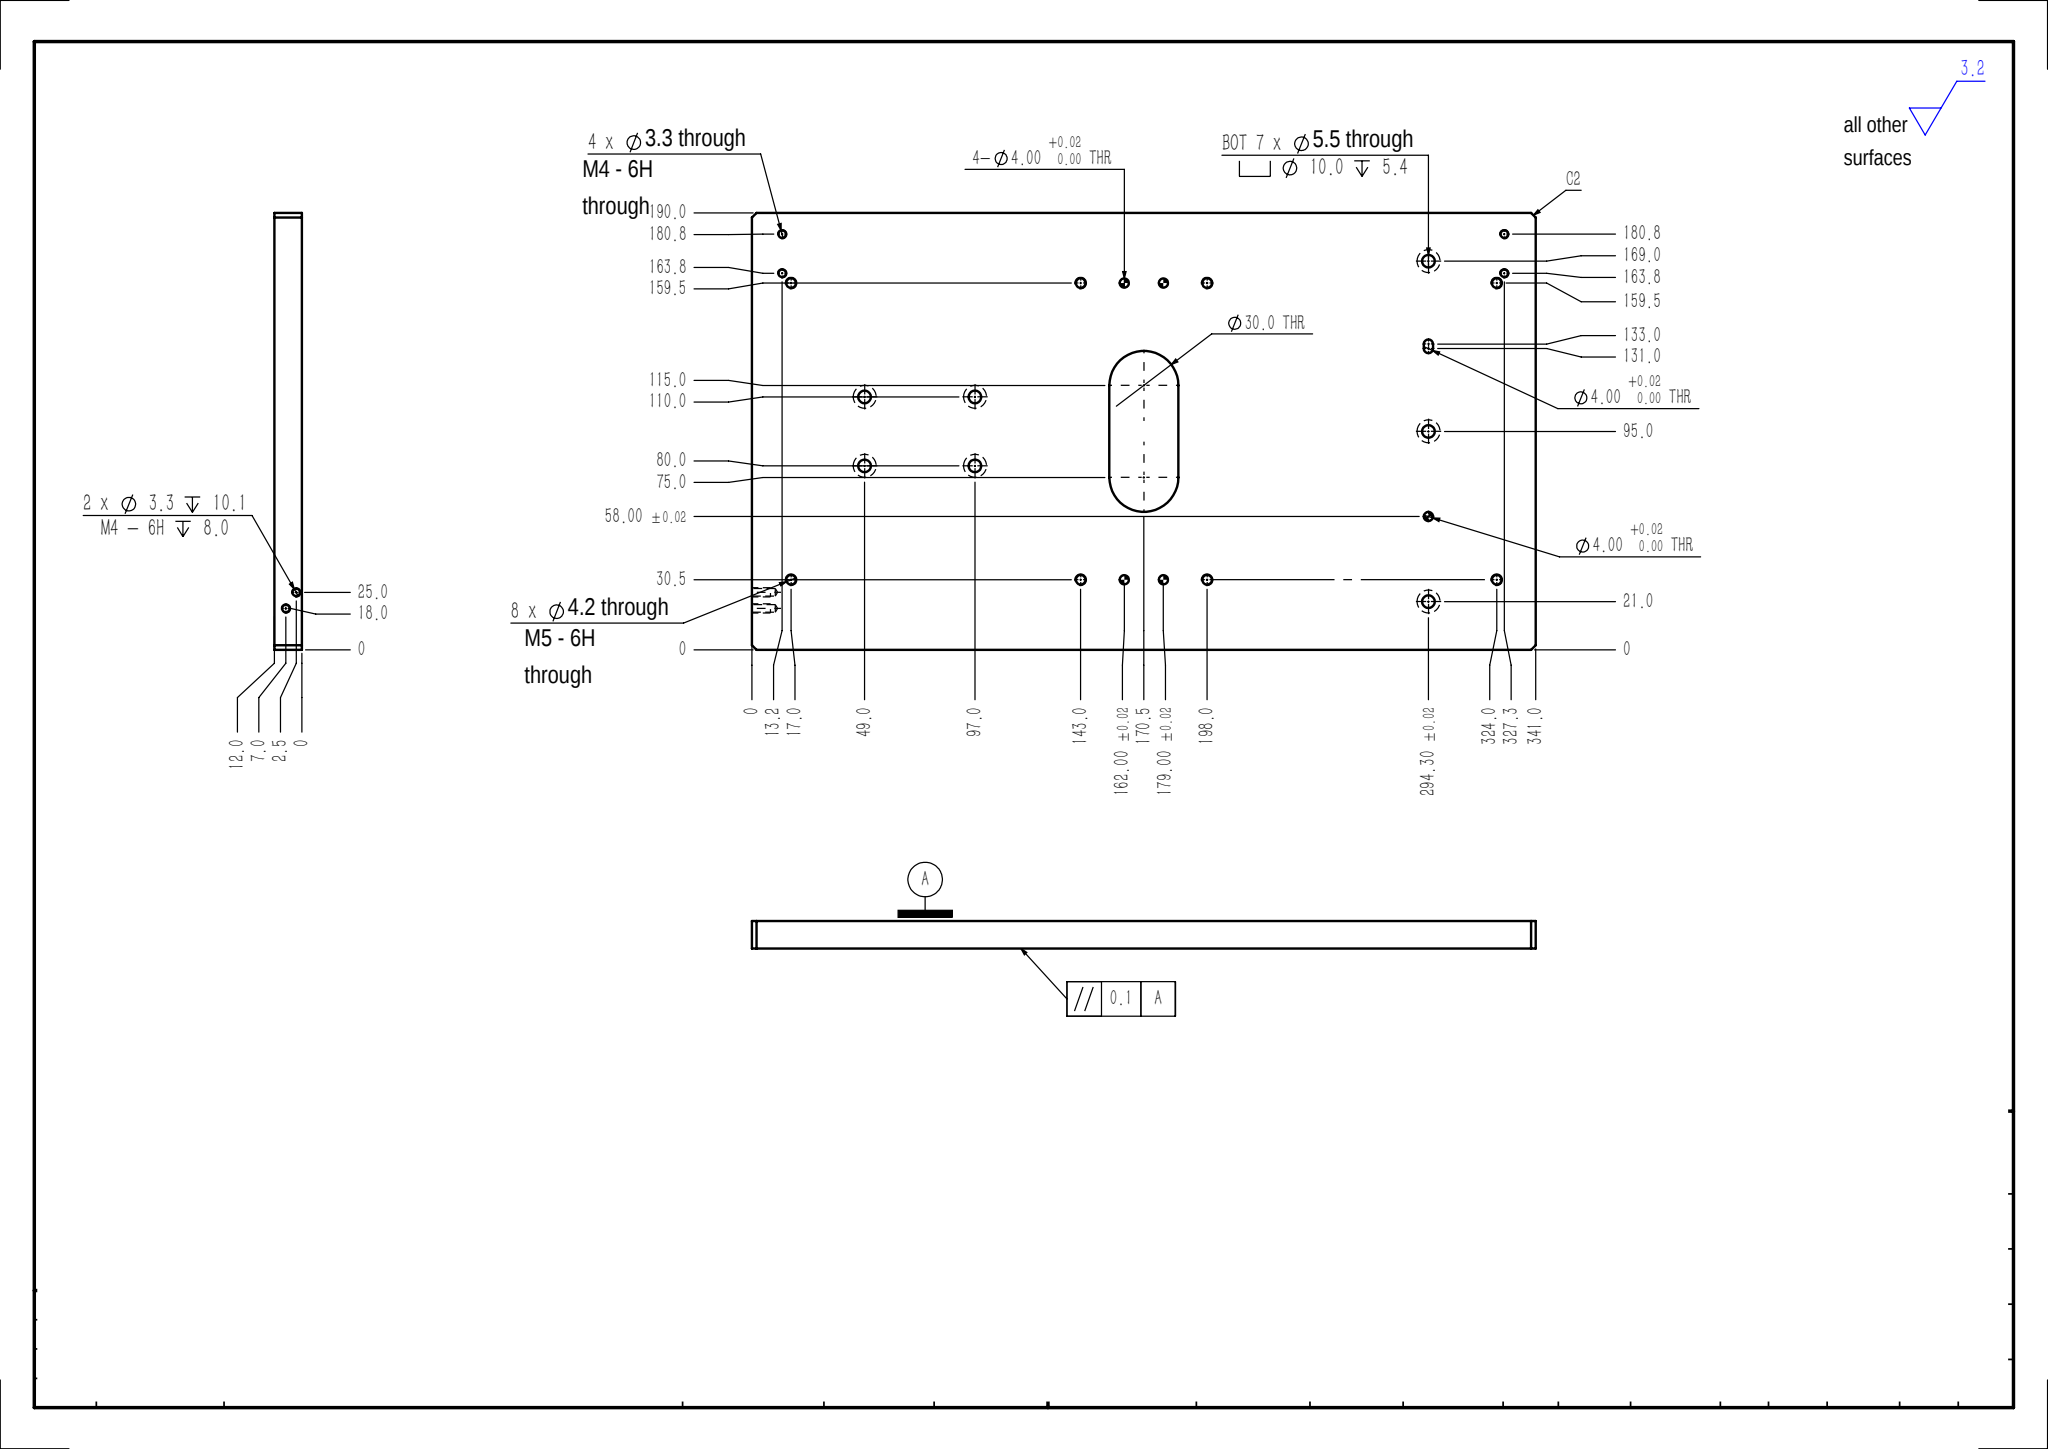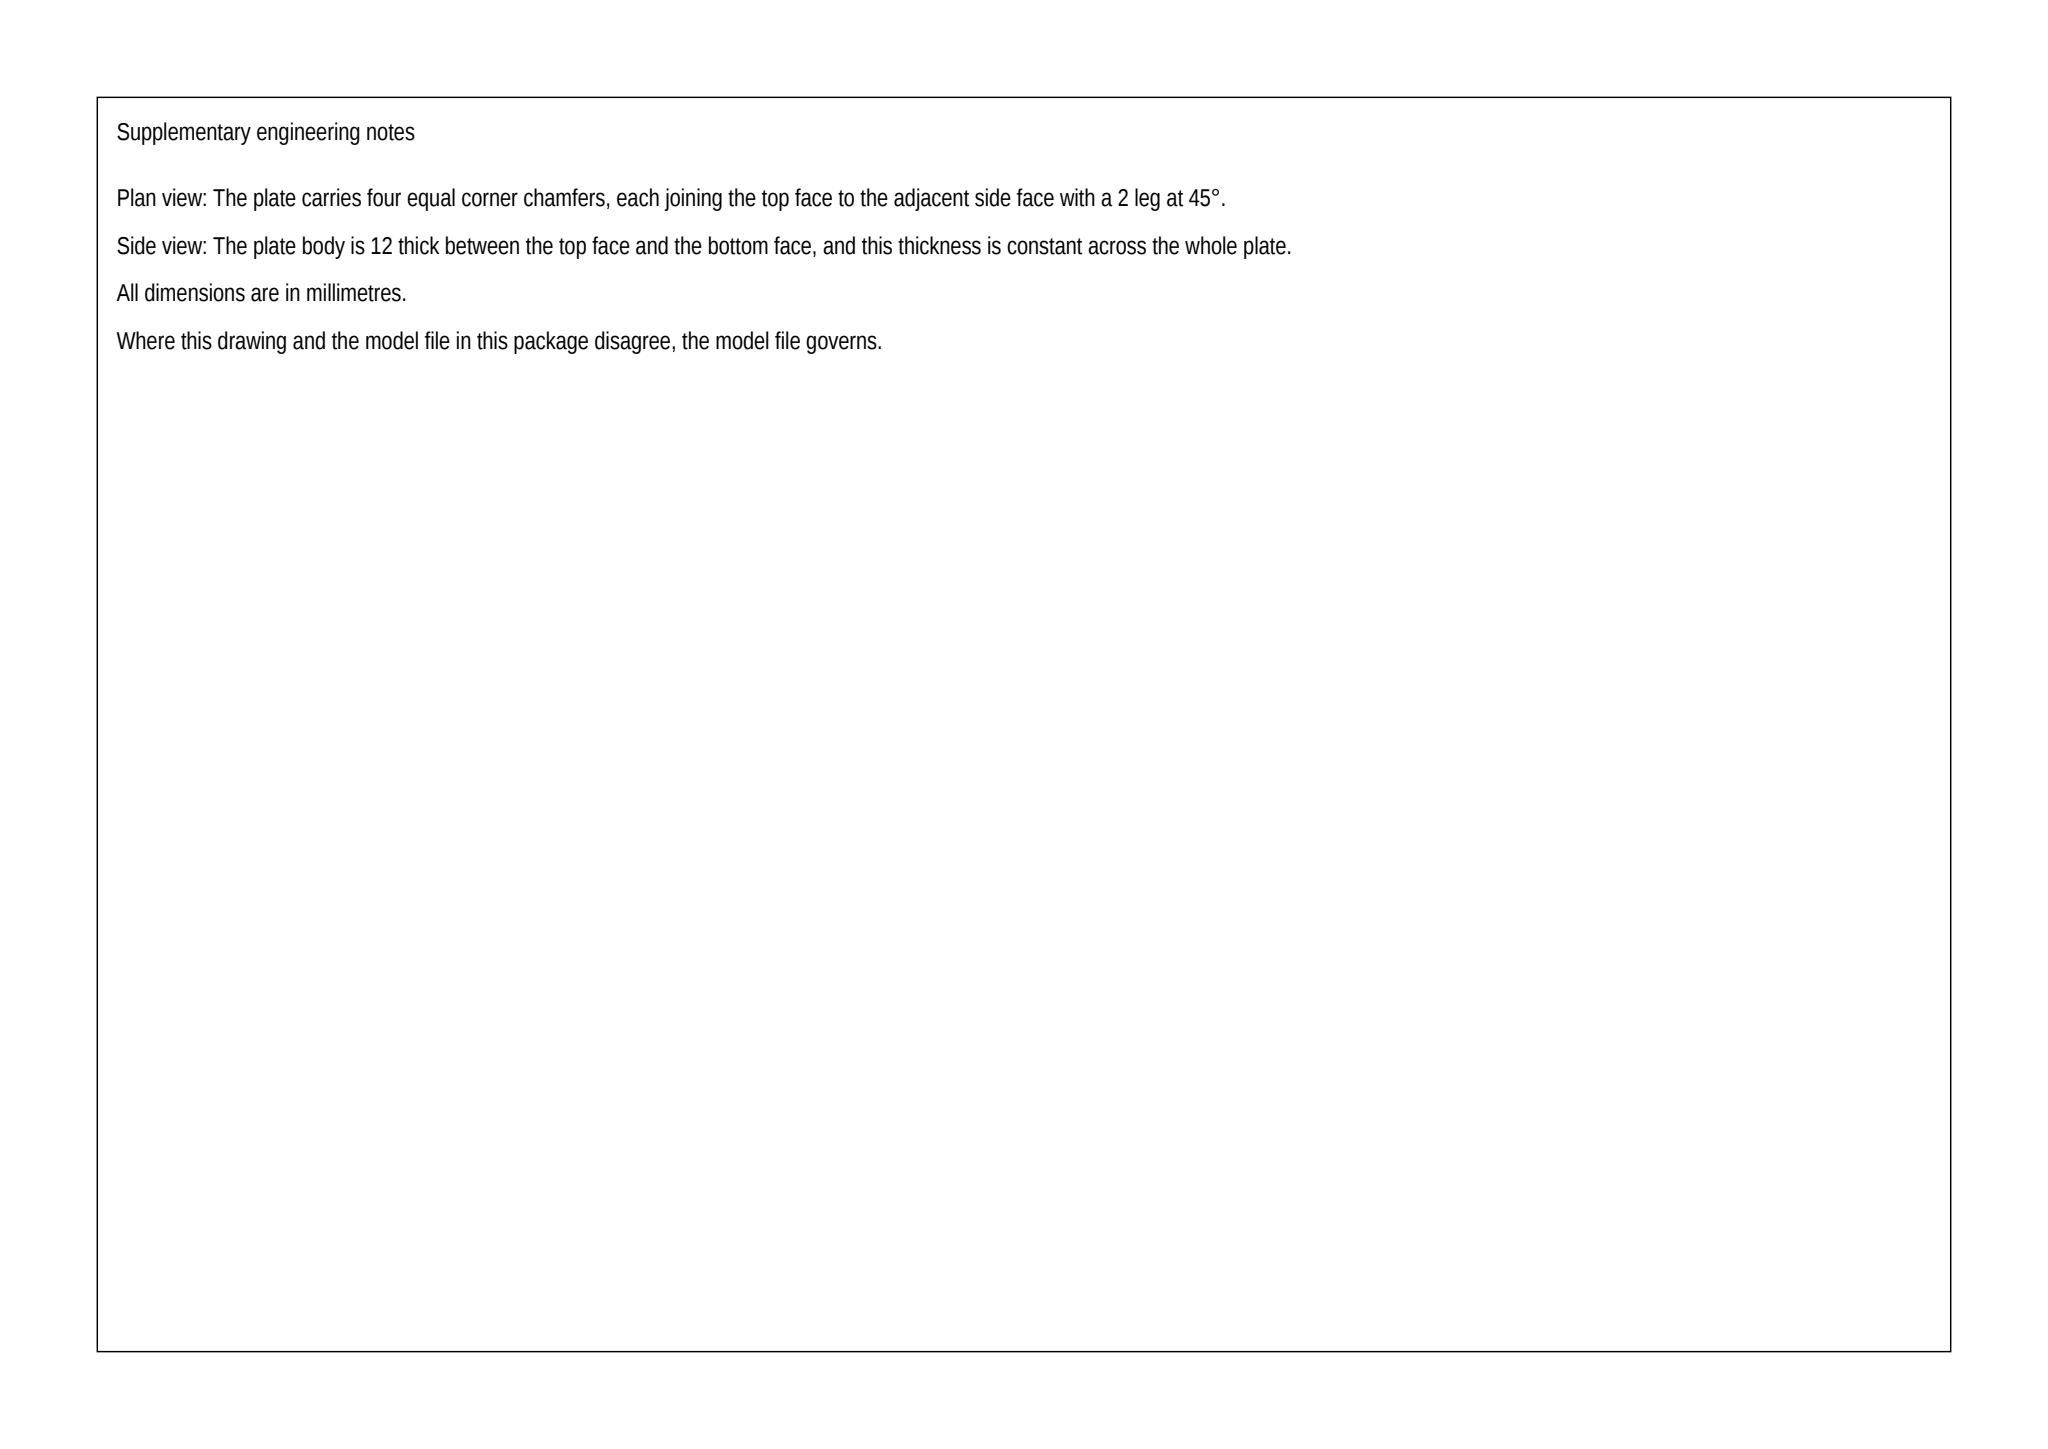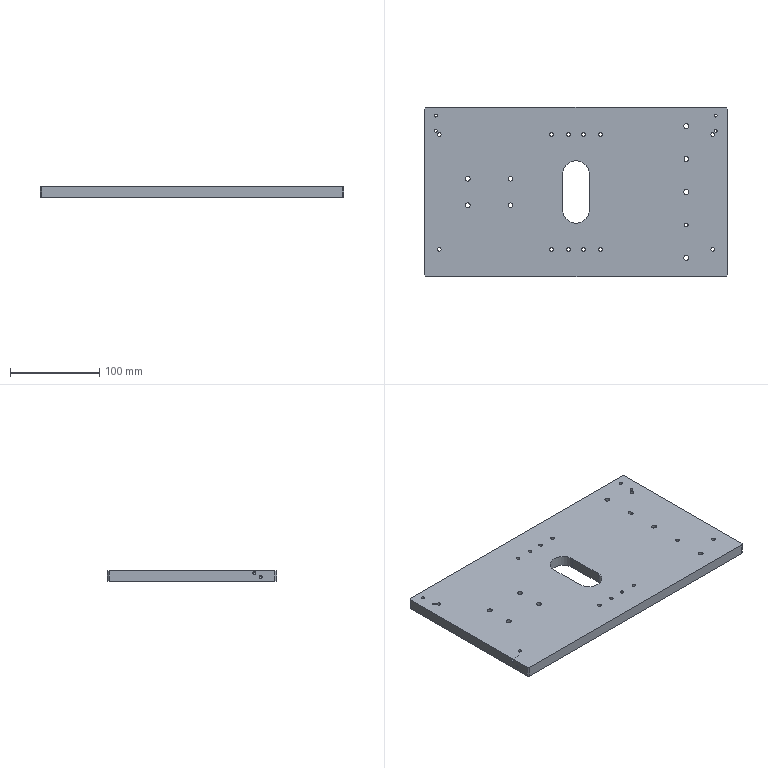Part | SolidWorks | mm | 1 solid | 95 faces | box 341 x 190 x 12 mm | volume 747515 mm3 | cylinder 70 | plane 21 | cone 4 | commonest cylinder face diameters 4.2 x16 10 x14 5.5 x14 3.3 x12 4 x12 30 x2
build123d program:
from build123d import *

# Parameters (mm, degrees)
SKETCH1_W                                       = 341
SKETCH1_H                                       = 190
BOSS_EXTRUDE1_DEPTH                             = 6
M5_HEX_SOCKET_HEAD_CAP_SCREW_CBORE1_D           = 5.5
M5_HEX_SOCKET_HEAD_CAP_SCREW_CBORE1_CBORE_D     = 10
M5_HEX_SOCKET_HEAD_CAP_SCREW_CBORE1_CBORE_DEPTH = 5.4
SKETCH5_R                                       = 2
CUT_EXTRUDE1_DEPTH                              = 196.549
M4_TAPPED_HOLE1_D                               = 3.3
SIZE_MM_DOWEL_HOLE1_D                           = 4
M5_TAPPED_HOLE1_D                               = 4.2
CHAMFER1_SIZE                                   = 2
CUT_EXTRUDE2_DEPTH                              = 196.549
M4_TAPPED_HOLE2_D                               = 3.3
M4_TAPPED_HOLE2_DEPTH                           = 10.1
M4_TAPPED_HOLE2_TIP                             = 0.9914


with BuildPart() as part:
    # Sketch1 → Boss-Extrude1 (new, symmetric)
    with BuildSketch(Plane.XY):
        Rectangle(SKETCH1_W, SKETCH1_H)
    extrude(amount=BOSS_EXTRUDE1_DEPTH, both=True)

    # M5 Hex Socket Head Cap Screw CBORE1 (through all)
    with Locations(Plane(origin=(0, 0, -6), x_dir=(-1, 0, 0), z_dir=(0, 0, -1))):
        with Locations((121.5, -15), (73.5, -15), (121.5, 15), (73.5, 15), (-123.8, -74), (-123.8, 0), (-123.8, 74)):
            CounterBoreHole(M5_HEX_SOCKET_HEAD_CAP_SCREW_CBORE1_D / 2, M5_HEX_SOCKET_HEAD_CAP_SCREW_CBORE1_CBORE_D / 2, M5_HEX_SOCKET_HEAD_CAP_SCREW_CBORE1_CBORE_DEPTH)

    # Sketch5 → Cut-Extrude1 (cut, through all)
    with BuildSketch(Plane(origin=(0, 0, -6), x_dir=(-1, 0, 0), z_dir=(0, 0, -1))):
        with Locations((-123.8, -37)):
            Circle(SKETCH5_R)
        with BuildLine():
            Line((-121.8, 38), (-121.8, 36))
            ThreePointArc((-121.8, 36), (-123.8, 34), (-125.8, 36))
            Line((-125.8, 36), (-125.8, 38))
            ThreePointArc((-125.8, 38), (-123.8, 40), (-121.8, 38))
        make_face()
    extrude(amount=-CUT_EXTRUDE1_DEPTH, mode=Mode.SUBTRACT)

    # M4 Tapped Hole1 (through all)
    with Locations(Plane.XY.offset(6)):
        with Locations((-157.35, 68.75), (-157.35, 85.75), (156.8, 68.75), (156.8, 85.75)):
            Hole(M4_TAPPED_HOLE1_D / 2)

    # Size mm Dowel Hole1 (through all)
    with Locations(Plane(origin=(0, 0, -6), x_dir=(-1, 0, 0), z_dir=(0, 0, -1))):
        with Locations((8.5, -64.5), (-8.5, -64.5), (8.5, 64.5), (-8.5, 64.5)):
            Hole(SIZE_MM_DOWEL_HOLE1_D / 2)

    # M5 Tapped Hole1 (through all)
    with Locations(Plane(origin=(0, 0, -6), x_dir=(-1, 0, 0), z_dir=(0, 0, -1))):
        with Locations((153.5, -64.5), (27.5, -64.5), (153.5, 64.5), (27.5, 64.5), (-27.5, 64.5), (-153.5, 64.5), (-27.5, -64.5), (-153.5, -64.5)):
            Hole(M5_TAPPED_HOLE1_D / 2)

    # Chamfer1
    chamfer1_edges = [part.edges().sort_by_distance(p)[0] for p in [
        (170.5, -95, 0),
        (-170.5, -95, 0),
        (-170.5, 95, 0),
        (170.5, 95, 0),
    ]]
    chamfer(chamfer1_edges, length=CHAMFER1_SIZE)

    # Sketch14 → Cut-Extrude2 (cut, through all)
    with BuildSketch(Plane(origin=(0, 0, -6), x_dir=(-1, 0, 0), z_dir=(0, 0, -1))):
        with BuildLine():
            Line((-15, -20), (-15, 20))
            ThreePointArc((-15, 20), (0, 35), (15, 20))
            Line((15, 20), (15, -20))
            ThreePointArc((15, -20), (0, -35), (-15, -20))
        make_face()
    extrude(amount=-CUT_EXTRUDE2_DEPTH, mode=Mode.SUBTRACT)

    # M4 Tapped Hole2
    with Locations(Plane.ZY.offset(170.5)):
        with Locations((-1, -77), (3.5, -70)):
            Hole(M4_TAPPED_HOLE2_D / 2, depth=M4_TAPPED_HOLE2_DEPTH)
            with Locations((0, 0, -(M4_TAPPED_HOLE2_DEPTH + M4_TAPPED_HOLE2_TIP / 2))):  # 118° drill point
                Cone(0, M4_TAPPED_HOLE2_D / 2, M4_TAPPED_HOLE2_TIP, mode=Mode.SUBTRACT)


solid = part.part